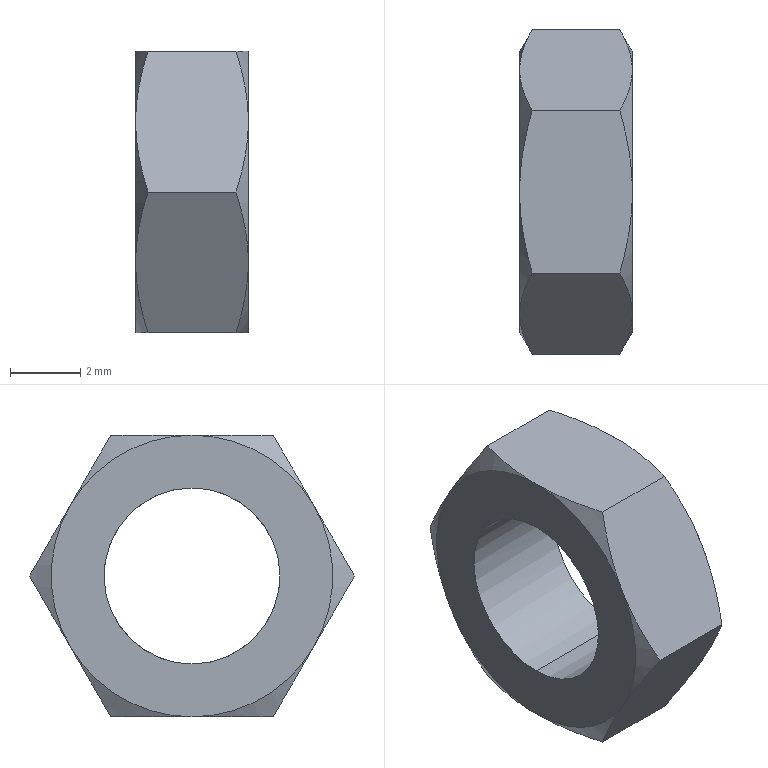Component | SolidWorks | USTH5-15-1_2-1 | 1 solid | 22 faces | box 3.2 x 9.24 x 8 mm | volume 113 mm3 | cone 12 | plane 8 | cylinder 2 | commonest cylinder face diameters 5 x2
STEP:
#1=COLOUR_RGB('',0.7922,0.8196,0.9333);
#2=FILL_AREA_STYLE_COLOUR('',#1);
#3=FILL_AREA_STYLE('',(#2));
#4=SURFACE_STYLE_FILL_AREA(#3);
#5=SURFACE_SIDE_STYLE('',(#4));
#6=SURFACE_STYLE_USAGE(.BOTH.,#5);
#7=PRESENTATION_STYLE_ASSIGNMENT((#6));
#8=CARTESIAN_POINT('',(19.157,0.9252,2.854));
#9=VERTEX_POINT('',#8);
#10=CARTESIAN_POINT('',(19.157,0.9252,3.051));
#11=VERTEX_POINT('',#10);
#12=CARTESIAN_POINT('',(19.157,0.9252,2.953));
#13=DIRECTION('',(-1.,0.,0.));
#14=DIRECTION('',(0.,0.,1.));
#15=AXIS2_PLACEMENT_3D('',#12,#13,#14);
#16=CIRCLE('',#15,0.09843);
#17=EDGE_CURVE('',#9,#11,#16,.T.);
#18=ORIENTED_EDGE('',*,*,#17,.F.);
#19=CARTESIAN_POINT('',(19.031,0.9252,2.854));
#20=VERTEX_POINT('',#19);
#21=CARTESIAN_POINT('',(19.157,0.9252,2.854));
#22=DIRECTION('',(-1.,0.,0.));
#23=VECTOR('',#22,39.37);
#24=LINE('',#21,#23);
#25=EDGE_CURVE('',#9,#20,#24,.T.);
#26=ORIENTED_EDGE('',*,*,#25,.T.);
#27=CARTESIAN_POINT('',(19.031,0.9252,3.051));
#28=VERTEX_POINT('',#27);
#29=CARTESIAN_POINT('',(19.031,0.9252,2.854));
#30=CARTESIAN_POINT('',(19.031,0.9123,2.854));
#31=CARTESIAN_POINT('',(19.031,0.8994,2.857));
#32=CARTESIAN_POINT('',(19.031,0.8756,2.867));
#33=CARTESIAN_POINT('',(19.031,0.8647,2.874));
#34=CARTESIAN_POINT('',(19.031,0.8465,2.892));
#35=CARTESIAN_POINT('',(19.031,0.8392,2.903));
#36=CARTESIAN_POINT('',(19.031,0.8293,2.927));
#37=CARTESIAN_POINT('',(19.031,0.8268,2.94));
#38=CARTESIAN_POINT('',(19.031,0.8268,2.966));
#39=CARTESIAN_POINT('',(19.031,0.8293,2.979));
#40=CARTESIAN_POINT('',(19.031,0.8392,3.002));
#41=CARTESIAN_POINT('',(19.031,0.8465,3.013));
#42=CARTESIAN_POINT('',(19.031,0.8647,3.031));
#43=CARTESIAN_POINT('',(19.031,0.8756,3.039));
#44=CARTESIAN_POINT('',(19.031,0.8994,3.049));
#45=CARTESIAN_POINT('',(19.031,0.9123,3.051));
#46=CARTESIAN_POINT('',(19.031,0.9252,3.051));
#47=B_SPLINE_CURVE_WITH_KNOTS('',3,(#29,#30,#31,#32,#33,#34,#35,#36,#37,#38,#39,#40,#41,#42,#43,#44,#45,#46),.UNSPECIFIED.,.F.,.F.,(4,2,2,2,2,2,2,2,4),(0.5,0.5625,0.625,0.6875,0.75,0.8125,0.875,0.9375,1.),.UNSPECIFIED.);
#48=EDGE_CURVE('',#20,#28,#47,.T.);
#49=ORIENTED_EDGE('',*,*,#48,.T.);
#50=CARTESIAN_POINT('',(19.157,0.9252,3.051));
#51=DIRECTION('',(-1.,0.,0.));
#52=VECTOR('',#51,39.37);
#53=LINE('',#50,#52);
#54=EDGE_CURVE('',#11,#28,#53,.T.);
#55=ORIENTED_EDGE('',*,*,#54,.F.);
#56=EDGE_LOOP('',(#18,#26,#49,#55));
#57=FACE_OUTER_BOUND('',#56,.T.);
#58=CARTESIAN_POINT('',(19.157,0.9252,2.953));
#59=DIRECTION('',(-1.,0.,0.));
#60=DIRECTION('',(0.,0.,1.));
#61=AXIS2_PLACEMENT_3D('',#58,#59,#60);
#62=CYLINDRICAL_SURFACE('',#61,0.09843);
#63=ADVANCED_FACE('',(#57),#62,.F.);
#64=CARTESIAN_POINT('',(19.157,1.062,3.031));
#65=VERTEX_POINT('',#64);
#66=CARTESIAN_POINT('',(19.157,0.9252,3.11));
#67=VERTEX_POINT('',#66);
#68=CARTESIAN_POINT('',(19.157,0.9252,2.953));
#69=DIRECTION('',(1.,0.,0.));
#70=DIRECTION('',(0.,0.,1.));
#71=AXIS2_PLACEMENT_3D('',#68,#69,#70);
#72=CIRCLE('',#71,0.1575);
#73=EDGE_CURVE('',#65,#67,#72,.T.);
#74=ORIENTED_EDGE('',*,*,#73,.T.);
#75=CARTESIAN_POINT('',(19.157,0.7888,3.031));
#76=VERTEX_POINT('',#75);
#77=CARTESIAN_POINT('',(19.157,0.9252,2.953));
#78=DIRECTION('',(1.,0.,0.));
#79=DIRECTION('',(0.,0.,1.));
#80=AXIS2_PLACEMENT_3D('',#77,#78,#79);
#81=CIRCLE('',#80,0.1575);
#82=EDGE_CURVE('',#67,#76,#81,.T.);
#83=ORIENTED_EDGE('',*,*,#82,.T.);
#84=CARTESIAN_POINT('',(19.157,0.7888,2.874));
#85=VERTEX_POINT('',#84);
#86=CARTESIAN_POINT('',(19.157,0.9252,2.953));
#87=DIRECTION('',(1.,0.,0.));
#88=DIRECTION('',(0.,0.,1.));
#89=AXIS2_PLACEMENT_3D('',#86,#87,#88);
#90=CIRCLE('',#89,0.1575);
#91=EDGE_CURVE('',#76,#85,#90,.T.);
#92=ORIENTED_EDGE('',*,*,#91,.T.);
#93=CARTESIAN_POINT('',(19.157,0.9252,2.795));
#94=VERTEX_POINT('',#93);
#95=CARTESIAN_POINT('',(19.157,0.9252,2.953));
#96=DIRECTION('',(1.,0.,0.));
#97=DIRECTION('',(0.,0.,1.));
#98=AXIS2_PLACEMENT_3D('',#95,#96,#97);
#99=CIRCLE('',#98,0.1575);
#100=EDGE_CURVE('',#85,#94,#99,.T.);
#101=ORIENTED_EDGE('',*,*,#100,.T.);
#102=CARTESIAN_POINT('',(19.157,1.062,2.874));
#103=VERTEX_POINT('',#102);
#104=CARTESIAN_POINT('',(19.157,0.9252,2.953));
#105=DIRECTION('',(1.,0.,0.));
#106=DIRECTION('',(0.,-0.,1.));
#107=AXIS2_PLACEMENT_3D('',#104,#105,#106);
#108=CIRCLE('',#107,0.1575);
#109=EDGE_CURVE('',#94,#103,#108,.T.);
#110=ORIENTED_EDGE('',*,*,#109,.T.);
#111=CARTESIAN_POINT('',(19.157,0.9252,2.953));
#112=DIRECTION('',(1.,0.,0.));
#113=DIRECTION('',(0.,0.,1.));
#114=AXIS2_PLACEMENT_3D('',#111,#112,#113);
#115=CIRCLE('',#114,0.1575);
#116=EDGE_CURVE('',#103,#65,#115,.T.);
#117=ORIENTED_EDGE('',*,*,#116,.T.);
#118=EDGE_LOOP('',(#74,#83,#92,#101,#110,#117));
#119=FACE_OUTER_BOUND('',#118,.T.);
#120=CARTESIAN_POINT('',(19.157,0.9252,2.953));
#121=DIRECTION('',(-1.,0.,0.));
#122=DIRECTION('',(0.,0.,1.));
#123=AXIS2_PLACEMENT_3D('',#120,#121,#122);
#124=CIRCLE('',#123,0.09843);
#125=EDGE_CURVE('',#11,#9,#124,.T.);
#126=ORIENTED_EDGE('',*,*,#125,.T.);
#127=ORIENTED_EDGE('',*,*,#17,.T.);
#128=EDGE_LOOP('',(#126,#127));
#129=FACE_BOUND('',#128,.T.);
#130=CARTESIAN_POINT('',(19.157,0.8465,2.953));
#131=DIRECTION('',(1.,0.,0.));
#132=DIRECTION('',(0.,0.,-1.));
#133=AXIS2_PLACEMENT_3D('',#130,#131,#132);
#134=PLANE('',#133);
#135=ADVANCED_FACE('',(#119,#129),#134,.T.);
#136=CARTESIAN_POINT('',(19.143,0.8343,3.11));
#137=VERTEX_POINT('',#136);
#138=CARTESIAN_POINT('',(19.143,0.8343,3.11));
#139=CARTESIAN_POINT('',(19.151,0.8194,3.085));
#140=CARTESIAN_POINT('',(19.157,0.8043,3.058));
#141=CARTESIAN_POINT('',(19.157,0.7888,3.031));
#142=B_SPLINE_CURVE_WITH_KNOTS('',3,(#138,#139,#140,#141),.UNSPECIFIED.,.F.,.F.,(4,4),(0.,0.002337),.UNSPECIFIED.);
#143=EDGE_CURVE('',#137,#76,#142,.T.);
#144=ORIENTED_EDGE('',*,*,#143,.T.);
#145=ORIENTED_EDGE('',*,*,#82,.F.);
#146=CARTESIAN_POINT('',(19.157,0.9252,3.11));
#147=CARTESIAN_POINT('',(19.157,0.8942,3.11));
#148=CARTESIAN_POINT('',(19.151,0.864,3.11));
#149=CARTESIAN_POINT('',(19.143,0.8343,3.11));
#150=B_SPLINE_CURVE_WITH_KNOTS('',3,(#146,#147,#148,#149),.UNSPECIFIED.,.F.,.F.,(4,4),(0.,0.002337),.UNSPECIFIED.);
#151=EDGE_CURVE('',#67,#137,#150,.T.);
#152=ORIENTED_EDGE('',*,*,#151,.T.);
#153=EDGE_LOOP('',(#144,#145,#152));
#154=FACE_OUTER_BOUND('',#153,.T.);
#155=CARTESIAN_POINT('',(19.143,0.9252,2.953));
#156=DIRECTION('',(-1.,0.,0.));
#157=DIRECTION('',(0.,0.,1.));
#158=AXIS2_PLACEMENT_3D('',#155,#156,#157);
#159=CONICAL_SURFACE('',#158,0.182,1.047);
#160=ADVANCED_FACE('',(#154),#159,.T.);
#161=CARTESIAN_POINT('',(19.143,1.016,3.11));
#162=VERTEX_POINT('',#161);
#163=CARTESIAN_POINT('',(19.143,1.016,3.11));
#164=CARTESIAN_POINT('',(19.151,0.9864,3.11));
#165=CARTESIAN_POINT('',(19.157,0.9562,3.11));
#166=CARTESIAN_POINT('',(19.157,0.9252,3.11));
#167=B_SPLINE_CURVE_WITH_KNOTS('',3,(#163,#164,#165,#166),.UNSPECIFIED.,.F.,.F.,(4,4),(0.,0.002337),.UNSPECIFIED.);
#168=EDGE_CURVE('',#162,#67,#167,.T.);
#169=ORIENTED_EDGE('',*,*,#168,.T.);
#170=ORIENTED_EDGE('',*,*,#73,.F.);
#171=CARTESIAN_POINT('',(19.157,1.062,3.031));
#172=CARTESIAN_POINT('',(19.157,1.046,3.058));
#173=CARTESIAN_POINT('',(19.151,1.031,3.085));
#174=CARTESIAN_POINT('',(19.143,1.016,3.11));
#175=B_SPLINE_CURVE_WITH_KNOTS('',3,(#171,#172,#173,#174),.UNSPECIFIED.,.F.,.F.,(4,4),(0.,0.002337),.UNSPECIFIED.);
#176=EDGE_CURVE('',#65,#162,#175,.T.);
#177=ORIENTED_EDGE('',*,*,#176,.T.);
#178=EDGE_LOOP('',(#169,#170,#177));
#179=FACE_OUTER_BOUND('',#178,.T.);
#180=CARTESIAN_POINT('',(19.143,0.9252,2.953));
#181=DIRECTION('',(-1.,0.,0.));
#182=DIRECTION('',(0.,0.,1.));
#183=AXIS2_PLACEMENT_3D('',#180,#181,#182);
#184=CONICAL_SURFACE('',#183,0.182,1.047);
#185=ADVANCED_FACE('',(#179),#184,.T.);
#186=CARTESIAN_POINT('',(19.143,1.107,2.953));
#187=VERTEX_POINT('',#186);
#188=CARTESIAN_POINT('',(19.143,1.107,2.953));
#189=CARTESIAN_POINT('',(19.151,1.092,2.978));
#190=CARTESIAN_POINT('',(19.157,1.077,3.005));
#191=CARTESIAN_POINT('',(19.157,1.062,3.031));
#192=B_SPLINE_CURVE_WITH_KNOTS('',3,(#188,#189,#190,#191),.UNSPECIFIED.,.F.,.F.,(4,4),(0.,0.002337),.UNSPECIFIED.);
#193=EDGE_CURVE('',#187,#65,#192,.T.);
#194=ORIENTED_EDGE('',*,*,#193,.T.);
#195=ORIENTED_EDGE('',*,*,#116,.F.);
#196=CARTESIAN_POINT('',(19.157,1.062,2.874));
#197=CARTESIAN_POINT('',(19.157,1.077,2.901));
#198=CARTESIAN_POINT('',(19.151,1.092,2.927));
#199=CARTESIAN_POINT('',(19.143,1.107,2.953));
#200=B_SPLINE_CURVE_WITH_KNOTS('',3,(#196,#197,#198,#199),.UNSPECIFIED.,.F.,.F.,(4,4),(0.,0.002337),.UNSPECIFIED.);
#201=EDGE_CURVE('',#103,#187,#200,.T.);
#202=ORIENTED_EDGE('',*,*,#201,.T.);
#203=EDGE_LOOP('',(#194,#195,#202));
#204=FACE_OUTER_BOUND('',#203,.T.);
#205=CARTESIAN_POINT('',(19.143,0.9252,2.953));
#206=DIRECTION('',(-1.,0.,0.));
#207=DIRECTION('',(0.,0.,1.));
#208=AXIS2_PLACEMENT_3D('',#205,#206,#207);
#209=CONICAL_SURFACE('',#208,0.182,1.047);
#210=ADVANCED_FACE('',(#204),#209,.T.);
#211=ORIENTED_EDGE('',*,*,#109,.F.);
#212=CARTESIAN_POINT('',(19.143,1.016,2.795));
#213=VERTEX_POINT('',#212);
#214=CARTESIAN_POINT('',(19.157,0.9252,2.795));
#215=CARTESIAN_POINT('',(19.157,0.9562,2.795));
#216=CARTESIAN_POINT('',(19.151,0.9864,2.795));
#217=CARTESIAN_POINT('',(19.143,1.016,2.795));
#218=B_SPLINE_CURVE_WITH_KNOTS('',3,(#214,#215,#216,#217),.UNSPECIFIED.,.F.,.F.,(4,4),(0.,0.002337),.UNSPECIFIED.);
#219=EDGE_CURVE('',#94,#213,#218,.T.);
#220=ORIENTED_EDGE('',*,*,#219,.T.);
#221=CARTESIAN_POINT('',(19.143,1.016,2.795));
#222=CARTESIAN_POINT('',(19.151,1.031,2.821));
#223=CARTESIAN_POINT('',(19.157,1.046,2.847));
#224=CARTESIAN_POINT('',(19.157,1.062,2.874));
#225=B_SPLINE_CURVE_WITH_KNOTS('',3,(#221,#222,#223,#224),.UNSPECIFIED.,.F.,.F.,(4,4),(0.,0.002337),.UNSPECIFIED.);
#226=EDGE_CURVE('',#213,#103,#225,.T.);
#227=ORIENTED_EDGE('',*,*,#226,.T.);
#228=EDGE_LOOP('',(#211,#220,#227));
#229=FACE_OUTER_BOUND('',#228,.T.);
#230=CARTESIAN_POINT('',(19.143,0.9252,2.953));
#231=DIRECTION('',(-1.,0.,0.));
#232=DIRECTION('',(0.,0.,1.));
#233=AXIS2_PLACEMENT_3D('',#230,#231,#232);
#234=CONICAL_SURFACE('',#233,0.182,1.047);
#235=ADVANCED_FACE('',(#229),#234,.T.);
#236=ORIENTED_EDGE('',*,*,#100,.F.);
#237=CARTESIAN_POINT('',(19.143,0.8343,2.795));
#238=VERTEX_POINT('',#237);
#239=CARTESIAN_POINT('',(19.157,0.7888,2.874));
#240=CARTESIAN_POINT('',(19.157,0.8043,2.847));
#241=CARTESIAN_POINT('',(19.151,0.8194,2.821));
#242=CARTESIAN_POINT('',(19.143,0.8343,2.795));
#243=B_SPLINE_CURVE_WITH_KNOTS('',3,(#239,#240,#241,#242),.UNSPECIFIED.,.F.,.F.,(4,4),(0.,0.002337),.UNSPECIFIED.);
#244=EDGE_CURVE('',#85,#238,#243,.T.);
#245=ORIENTED_EDGE('',*,*,#244,.T.);
#246=CARTESIAN_POINT('',(19.143,0.8343,2.795));
#247=CARTESIAN_POINT('',(19.151,0.864,2.795));
#248=CARTESIAN_POINT('',(19.157,0.8942,2.795));
#249=CARTESIAN_POINT('',(19.157,0.9252,2.795));
#250=B_SPLINE_CURVE_WITH_KNOTS('',3,(#246,#247,#248,#249),.UNSPECIFIED.,.F.,.F.,(4,4),(0.,0.002337),.UNSPECIFIED.);
#251=EDGE_CURVE('',#238,#94,#250,.T.);
#252=ORIENTED_EDGE('',*,*,#251,.T.);
#253=EDGE_LOOP('',(#236,#245,#252));
#254=FACE_OUTER_BOUND('',#253,.T.);
#255=CARTESIAN_POINT('',(19.143,0.9252,2.953));
#256=DIRECTION('',(-1.,0.,0.));
#257=DIRECTION('',(0.,0.,1.));
#258=AXIS2_PLACEMENT_3D('',#255,#256,#257);
#259=CONICAL_SURFACE('',#258,0.182,1.047);
#260=ADVANCED_FACE('',(#254),#259,.T.);
#261=CARTESIAN_POINT('',(19.143,0.7434,2.953));
#262=VERTEX_POINT('',#261);
#263=CARTESIAN_POINT('',(19.143,0.7434,2.953));
#264=CARTESIAN_POINT('',(19.151,0.7582,2.927));
#265=CARTESIAN_POINT('',(19.157,0.7733,2.901));
#266=CARTESIAN_POINT('',(19.157,0.7888,2.874));
#267=B_SPLINE_CURVE_WITH_KNOTS('',3,(#263,#264,#265,#266),.UNSPECIFIED.,.F.,.F.,(4,4),(0.,0.002337),.UNSPECIFIED.);
#268=EDGE_CURVE('',#262,#85,#267,.T.);
#269=ORIENTED_EDGE('',*,*,#268,.T.);
#270=ORIENTED_EDGE('',*,*,#91,.F.);
#271=CARTESIAN_POINT('',(19.157,0.7888,3.031));
#272=CARTESIAN_POINT('',(19.157,0.7733,3.005));
#273=CARTESIAN_POINT('',(19.151,0.7582,2.978));
#274=CARTESIAN_POINT('',(19.143,0.7434,2.953));
#275=B_SPLINE_CURVE_WITH_KNOTS('',3,(#271,#272,#273,#274),.UNSPECIFIED.,.F.,.F.,(4,4),(0.,0.002337),.UNSPECIFIED.);
#276=EDGE_CURVE('',#76,#262,#275,.T.);
#277=ORIENTED_EDGE('',*,*,#276,.T.);
#278=EDGE_LOOP('',(#269,#270,#277));
#279=FACE_OUTER_BOUND('',#278,.T.);
#280=CARTESIAN_POINT('',(19.143,0.9252,2.953));
#281=DIRECTION('',(-1.,0.,0.));
#282=DIRECTION('',(0.,0.,1.));
#283=AXIS2_PLACEMENT_3D('',#280,#281,#282);
#284=CONICAL_SURFACE('',#283,0.182,1.047);
#285=ADVANCED_FACE('',(#279),#284,.T.);
#286=CARTESIAN_POINT('',(19.045,0.8343,3.11));
#287=VERTEX_POINT('',#286);
#288=CARTESIAN_POINT('',(18.968,0.8343,3.11));
#289=DIRECTION('',(1.,0.,0.));
#290=VECTOR('',#289,39.37);
#291=LINE('',#288,#290);
#292=EDGE_CURVE('',#287,#137,#291,.T.);
#293=ORIENTED_EDGE('',*,*,#292,.F.);
#294=CARTESIAN_POINT('',(19.031,0.7888,3.031));
#295=VERTEX_POINT('',#294);
#296=CARTESIAN_POINT('',(19.031,0.7888,3.031));
#297=CARTESIAN_POINT('',(19.031,0.8043,3.058));
#298=CARTESIAN_POINT('',(19.036,0.8194,3.085));
#299=CARTESIAN_POINT('',(19.045,0.8343,3.11));
#300=B_SPLINE_CURVE_WITH_KNOTS('',3,(#296,#297,#298,#299),.UNSPECIFIED.,.F.,.F.,(4,4),(0.,0.002337),.UNSPECIFIED.);
#301=EDGE_CURVE('',#295,#287,#300,.T.);
#302=ORIENTED_EDGE('',*,*,#301,.F.);
#303=CARTESIAN_POINT('',(19.045,0.7434,2.953));
#304=VERTEX_POINT('',#303);
#305=CARTESIAN_POINT('',(19.045,0.7434,2.953));
#306=CARTESIAN_POINT('',(19.036,0.7582,2.978));
#307=CARTESIAN_POINT('',(19.031,0.7733,3.005));
#308=CARTESIAN_POINT('',(19.031,0.7888,3.031));
#309=B_SPLINE_CURVE_WITH_KNOTS('',3,(#305,#306,#307,#308),.UNSPECIFIED.,.F.,.F.,(4,4),(0.,0.002337),.UNSPECIFIED.);
#310=EDGE_CURVE('',#304,#295,#309,.T.);
#311=ORIENTED_EDGE('',*,*,#310,.F.);
#312=CARTESIAN_POINT('',(18.968,0.7434,2.953));
#313=DIRECTION('',(-1.,0.,0.));
#314=VECTOR('',#313,39.37);
#315=LINE('',#312,#314);
#316=EDGE_CURVE('',#262,#304,#315,.T.);
#317=ORIENTED_EDGE('',*,*,#316,.F.);
#318=ORIENTED_EDGE('',*,*,#276,.F.);
#319=ORIENTED_EDGE('',*,*,#143,.F.);
#320=EDGE_LOOP('',(#293,#302,#311,#317,#318,#319));
#321=FACE_OUTER_BOUND('',#320,.T.);
#322=CARTESIAN_POINT('',(18.968,0.8343,3.11));
#323=DIRECTION('',(0.,0.866,-0.5));
#324=DIRECTION('',(0.,0.5,0.866));
#325=AXIS2_PLACEMENT_3D('',#322,#323,#324);
#326=PLANE('',#325);
#327=ADVANCED_FACE('',(#321),#326,.F.);
#328=CARTESIAN_POINT('',(19.045,1.016,3.11));
#329=VERTEX_POINT('',#328);
#330=CARTESIAN_POINT('',(18.968,1.016,3.11));
#331=DIRECTION('',(1.,0.,0.));
#332=VECTOR('',#331,39.37);
#333=LINE('',#330,#332);
#334=EDGE_CURVE('',#329,#162,#333,.T.);
#335=ORIENTED_EDGE('',*,*,#334,.F.);
#336=CARTESIAN_POINT('',(19.031,0.9252,3.11));
#337=VERTEX_POINT('',#336);
#338=CARTESIAN_POINT('',(19.031,0.9252,3.11));
#339=CARTESIAN_POINT('',(19.031,0.9562,3.11));
#340=CARTESIAN_POINT('',(19.036,0.9864,3.11));
#341=CARTESIAN_POINT('',(19.045,1.016,3.11));
#342=B_SPLINE_CURVE_WITH_KNOTS('',3,(#338,#339,#340,#341),.UNSPECIFIED.,.F.,.F.,(4,4),(0.,0.002337),.UNSPECIFIED.);
#343=EDGE_CURVE('',#337,#329,#342,.T.);
#344=ORIENTED_EDGE('',*,*,#343,.F.);
#345=CARTESIAN_POINT('',(19.045,0.8343,3.11));
#346=CARTESIAN_POINT('',(19.036,0.864,3.11));
#347=CARTESIAN_POINT('',(19.031,0.8942,3.11));
#348=CARTESIAN_POINT('',(19.031,0.9252,3.11));
#349=B_SPLINE_CURVE_WITH_KNOTS('',3,(#345,#346,#347,#348),.UNSPECIFIED.,.F.,.F.,(4,4),(0.,0.002337),.UNSPECIFIED.);
#350=EDGE_CURVE('',#287,#337,#349,.T.);
#351=ORIENTED_EDGE('',*,*,#350,.F.);
#352=ORIENTED_EDGE('',*,*,#292,.T.);
#353=ORIENTED_EDGE('',*,*,#151,.F.);
#354=ORIENTED_EDGE('',*,*,#168,.F.);
#355=EDGE_LOOP('',(#335,#344,#351,#352,#353,#354));
#356=FACE_OUTER_BOUND('',#355,.T.);
#357=CARTESIAN_POINT('',(18.968,1.016,3.11));
#358=DIRECTION('',(0.,0.,-1.));
#359=DIRECTION('',(-1.,0.,0.));
#360=AXIS2_PLACEMENT_3D('',#357,#358,#359);
#361=PLANE('',#360);
#362=ADVANCED_FACE('',(#356),#361,.F.);
#363=CARTESIAN_POINT('',(19.045,1.107,2.953));
#364=VERTEX_POINT('',#363);
#365=CARTESIAN_POINT('',(18.968,1.107,2.953));
#366=DIRECTION('',(1.,0.,0.));
#367=VECTOR('',#366,39.37);
#368=LINE('',#365,#367);
#369=EDGE_CURVE('',#364,#187,#368,.T.);
#370=ORIENTED_EDGE('',*,*,#369,.F.);
#371=CARTESIAN_POINT('',(19.031,1.062,3.031));
#372=VERTEX_POINT('',#371);
#373=CARTESIAN_POINT('',(19.031,1.062,3.031));
#374=CARTESIAN_POINT('',(19.031,1.077,3.005));
#375=CARTESIAN_POINT('',(19.036,1.092,2.978));
#376=CARTESIAN_POINT('',(19.045,1.107,2.953));
#377=B_SPLINE_CURVE_WITH_KNOTS('',3,(#373,#374,#375,#376),.UNSPECIFIED.,.F.,.F.,(4,4),(0.,0.002337),.UNSPECIFIED.);
#378=EDGE_CURVE('',#372,#364,#377,.T.);
#379=ORIENTED_EDGE('',*,*,#378,.F.);
#380=CARTESIAN_POINT('',(19.045,1.016,3.11));
#381=CARTESIAN_POINT('',(19.036,1.031,3.085));
#382=CARTESIAN_POINT('',(19.031,1.046,3.058));
#383=CARTESIAN_POINT('',(19.031,1.062,3.031));
#384=B_SPLINE_CURVE_WITH_KNOTS('',3,(#380,#381,#382,#383),.UNSPECIFIED.,.F.,.F.,(4,4),(0.,0.002337),.UNSPECIFIED.);
#385=EDGE_CURVE('',#329,#372,#384,.T.);
#386=ORIENTED_EDGE('',*,*,#385,.F.);
#387=ORIENTED_EDGE('',*,*,#334,.T.);
#388=ORIENTED_EDGE('',*,*,#176,.F.);
#389=ORIENTED_EDGE('',*,*,#193,.F.);
#390=EDGE_LOOP('',(#370,#379,#386,#387,#388,#389));
#391=FACE_OUTER_BOUND('',#390,.T.);
#392=CARTESIAN_POINT('',(18.968,1.107,2.953));
#393=DIRECTION('',(0.,-0.866,-0.5));
#394=DIRECTION('',(0.,0.5,-0.866));
#395=AXIS2_PLACEMENT_3D('',#392,#393,#394);
#396=PLANE('',#395);
#397=ADVANCED_FACE('',(#391),#396,.F.);
#398=ORIENTED_EDGE('',*,*,#226,.F.);
#399=CARTESIAN_POINT('',(19.045,1.016,2.795));
#400=VERTEX_POINT('',#399);
#401=CARTESIAN_POINT('',(18.968,1.016,2.795));
#402=DIRECTION('',(1.,0.,0.));
#403=VECTOR('',#402,39.37);
#404=LINE('',#401,#403);
#405=EDGE_CURVE('',#400,#213,#404,.T.);
#406=ORIENTED_EDGE('',*,*,#405,.F.);
#407=CARTESIAN_POINT('',(19.031,1.062,2.874));
#408=VERTEX_POINT('',#407);
#409=CARTESIAN_POINT('',(19.031,1.062,2.874));
#410=CARTESIAN_POINT('',(19.031,1.046,2.847));
#411=CARTESIAN_POINT('',(19.036,1.031,2.821));
#412=CARTESIAN_POINT('',(19.045,1.016,2.795));
#413=B_SPLINE_CURVE_WITH_KNOTS('',3,(#409,#410,#411,#412),.UNSPECIFIED.,.F.,.F.,(4,4),(0.,0.002337),.UNSPECIFIED.);
#414=EDGE_CURVE('',#408,#400,#413,.T.);
#415=ORIENTED_EDGE('',*,*,#414,.F.);
#416=CARTESIAN_POINT('',(19.045,1.107,2.953));
#417=CARTESIAN_POINT('',(19.036,1.092,2.927));
#418=CARTESIAN_POINT('',(19.031,1.077,2.901));
#419=CARTESIAN_POINT('',(19.031,1.062,2.874));
#420=B_SPLINE_CURVE_WITH_KNOTS('',3,(#416,#417,#418,#419),.UNSPECIFIED.,.F.,.F.,(4,4),(0.,0.002337),.UNSPECIFIED.);
#421=EDGE_CURVE('',#364,#408,#420,.T.);
#422=ORIENTED_EDGE('',*,*,#421,.F.);
#423=ORIENTED_EDGE('',*,*,#369,.T.);
#424=ORIENTED_EDGE('',*,*,#201,.F.);
#425=EDGE_LOOP('',(#398,#406,#415,#422,#423,#424));
#426=FACE_OUTER_BOUND('',#425,.T.);
#427=CARTESIAN_POINT('',(18.968,1.016,2.795));
#428=DIRECTION('',(0.,-0.866,0.5));
#429=DIRECTION('',(0.,-0.5,-0.866));
#430=AXIS2_PLACEMENT_3D('',#427,#428,#429);
#431=PLANE('',#430);
#432=ADVANCED_FACE('',(#426),#431,.F.);
#433=ORIENTED_EDGE('',*,*,#251,.F.);
#434=CARTESIAN_POINT('',(19.045,0.8343,2.795));
#435=VERTEX_POINT('',#434);
#436=CARTESIAN_POINT('',(18.968,0.8343,2.795));
#437=DIRECTION('',(1.,0.,0.));
#438=VECTOR('',#437,39.37);
#439=LINE('',#436,#438);
#440=EDGE_CURVE('',#435,#238,#439,.T.);
#441=ORIENTED_EDGE('',*,*,#440,.F.);
#442=CARTESIAN_POINT('',(19.031,0.9252,2.795));
#443=VERTEX_POINT('',#442);
#444=CARTESIAN_POINT('',(19.031,0.9252,2.795));
#445=CARTESIAN_POINT('',(19.031,0.8942,2.795));
#446=CARTESIAN_POINT('',(19.036,0.864,2.795));
#447=CARTESIAN_POINT('',(19.045,0.8343,2.795));
#448=B_SPLINE_CURVE_WITH_KNOTS('',3,(#444,#445,#446,#447),.UNSPECIFIED.,.F.,.F.,(4,4),(0.,0.002337),.UNSPECIFIED.);
#449=EDGE_CURVE('',#443,#435,#448,.T.);
#450=ORIENTED_EDGE('',*,*,#449,.F.);
#451=CARTESIAN_POINT('',(19.045,1.016,2.795));
#452=CARTESIAN_POINT('',(19.036,0.9864,2.795));
#453=CARTESIAN_POINT('',(19.031,0.9562,2.795));
#454=CARTESIAN_POINT('',(19.031,0.9252,2.795));
#455=B_SPLINE_CURVE_WITH_KNOTS('',3,(#451,#452,#453,#454),.UNSPECIFIED.,.F.,.F.,(4,4),(0.,0.002337),.UNSPECIFIED.);
#456=EDGE_CURVE('',#400,#443,#455,.T.);
#457=ORIENTED_EDGE('',*,*,#456,.F.);
#458=ORIENTED_EDGE('',*,*,#405,.T.);
#459=ORIENTED_EDGE('',*,*,#219,.F.);
#460=EDGE_LOOP('',(#433,#441,#450,#457,#458,#459));
#461=FACE_OUTER_BOUND('',#460,.T.);
#462=CARTESIAN_POINT('',(18.968,0.8343,2.795));
#463=DIRECTION('',(0.,0.,1.));
#464=DIRECTION('',(1.,0.,0.));
#465=AXIS2_PLACEMENT_3D('',#462,#463,#464);
#466=PLANE('',#465);
#467=ADVANCED_FACE('',(#461),#466,.F.);
#468=ORIENTED_EDGE('',*,*,#268,.F.);
#469=ORIENTED_EDGE('',*,*,#316,.T.);
#470=CARTESIAN_POINT('',(19.031,0.7888,2.874));
#471=VERTEX_POINT('',#470);
#472=CARTESIAN_POINT('',(19.031,0.7888,2.874));
#473=CARTESIAN_POINT('',(19.031,0.7733,2.901));
#474=CARTESIAN_POINT('',(19.036,0.7582,2.927));
#475=CARTESIAN_POINT('',(19.045,0.7434,2.953));
#476=B_SPLINE_CURVE_WITH_KNOTS('',3,(#472,#473,#474,#475),.UNSPECIFIED.,.F.,.F.,(4,4),(0.,0.002337),.UNSPECIFIED.);
#477=EDGE_CURVE('',#471,#304,#476,.T.);
#478=ORIENTED_EDGE('',*,*,#477,.F.);
#479=CARTESIAN_POINT('',(19.045,0.8343,2.795));
#480=CARTESIAN_POINT('',(19.036,0.8194,2.821));
#481=CARTESIAN_POINT('',(19.031,0.8043,2.847));
#482=CARTESIAN_POINT('',(19.031,0.7888,2.874));
#483=B_SPLINE_CURVE_WITH_KNOTS('',3,(#479,#480,#481,#482),.UNSPECIFIED.,.F.,.F.,(4,4),(0.,0.002337),.UNSPECIFIED.);
#484=EDGE_CURVE('',#435,#471,#483,.T.);
#485=ORIENTED_EDGE('',*,*,#484,.F.);
#486=ORIENTED_EDGE('',*,*,#440,.T.);
#487=ORIENTED_EDGE('',*,*,#244,.F.);
#488=EDGE_LOOP('',(#468,#469,#478,#485,#486,#487));
#489=FACE_OUTER_BOUND('',#488,.T.);
#490=CARTESIAN_POINT('',(18.968,0.7434,2.953));
#491=DIRECTION('',(0.,0.866,0.5));
#492=DIRECTION('',(0.,-0.5,0.866));
#493=AXIS2_PLACEMENT_3D('',#490,#491,#492);
#494=PLANE('',#493);
#495=ADVANCED_FACE('',(#489),#494,.F.);
#496=ORIENTED_EDGE('',*,*,#350,.T.);
#497=CARTESIAN_POINT('',(19.031,0.9252,2.953));
#498=DIRECTION('',(1.,0.,0.));
#499=DIRECTION('',(0.,0.,-1.));
#500=AXIS2_PLACEMENT_3D('',#497,#498,#499);
#501=CIRCLE('',#500,0.1575);
#502=EDGE_CURVE('',#337,#295,#501,.T.);
#503=ORIENTED_EDGE('',*,*,#502,.T.);
#504=ORIENTED_EDGE('',*,*,#301,.T.);
#505=EDGE_LOOP('',(#496,#503,#504));
#506=FACE_OUTER_BOUND('',#505,.T.);
#507=CARTESIAN_POINT('',(19.045,0.9252,2.953));
#508=DIRECTION('',(1.,0.,0.));
#509=DIRECTION('',(0.,0.,-1.));
#510=AXIS2_PLACEMENT_3D('',#507,#508,#509);
#511=CONICAL_SURFACE('',#510,0.182,1.047);
#512=ADVANCED_FACE('',(#506),#511,.T.);
#513=ORIENTED_EDGE('',*,*,#310,.T.);
#514=CARTESIAN_POINT('',(19.031,0.9252,2.953));
#515=DIRECTION('',(1.,0.,0.));
#516=DIRECTION('',(0.,0.,-1.));
#517=AXIS2_PLACEMENT_3D('',#514,#515,#516);
#518=CIRCLE('',#517,0.1575);
#519=EDGE_CURVE('',#295,#471,#518,.T.);
#520=ORIENTED_EDGE('',*,*,#519,.T.);
#521=ORIENTED_EDGE('',*,*,#477,.T.);
#522=EDGE_LOOP('',(#513,#520,#521));
#523=FACE_OUTER_BOUND('',#522,.T.);
#524=CARTESIAN_POINT('',(19.045,0.9252,2.953));
#525=DIRECTION('',(1.,0.,0.));
#526=DIRECTION('',(0.,0.,-1.));
#527=AXIS2_PLACEMENT_3D('',#524,#525,#526);
#528=CONICAL_SURFACE('',#527,0.182,1.047);
#529=ADVANCED_FACE('',(#523),#528,.T.);
#530=CARTESIAN_POINT('',(19.031,0.9252,2.953));
#531=DIRECTION('',(1.,0.,0.));
#532=DIRECTION('',(0.,0.,-1.));
#533=AXIS2_PLACEMENT_3D('',#530,#531,#532);
#534=CIRCLE('',#533,0.1575);
#535=EDGE_CURVE('',#372,#337,#534,.T.);
#536=ORIENTED_EDGE('',*,*,#535,.T.);
#537=ORIENTED_EDGE('',*,*,#343,.T.);
#538=ORIENTED_EDGE('',*,*,#385,.T.);
#539=EDGE_LOOP('',(#536,#537,#538));
#540=FACE_OUTER_BOUND('',#539,.T.);
#541=CARTESIAN_POINT('',(19.045,0.9252,2.953));
#542=DIRECTION('',(1.,0.,0.));
#543=DIRECTION('',(0.,0.,-1.));
#544=AXIS2_PLACEMENT_3D('',#541,#542,#543);
#545=CONICAL_SURFACE('',#544,0.182,1.047);
#546=ADVANCED_FACE('',(#540),#545,.T.);
#547=CARTESIAN_POINT('',(19.031,0.9252,2.953));
#548=DIRECTION('',(1.,0.,0.));
#549=DIRECTION('',(0.,0.,-1.));
#550=AXIS2_PLACEMENT_3D('',#547,#548,#549);
#551=CIRCLE('',#550,0.1575);
#552=EDGE_CURVE('',#408,#372,#551,.T.);
#553=ORIENTED_EDGE('',*,*,#552,.T.);
#554=ORIENTED_EDGE('',*,*,#378,.T.);
#555=ORIENTED_EDGE('',*,*,#421,.T.);
#556=EDGE_LOOP('',(#553,#554,#555));
#557=FACE_OUTER_BOUND('',#556,.T.);
#558=CARTESIAN_POINT('',(19.045,0.9252,2.953));
#559=DIRECTION('',(1.,0.,0.));
#560=DIRECTION('',(0.,0.,-1.));
#561=AXIS2_PLACEMENT_3D('',#558,#559,#560);
#562=CONICAL_SURFACE('',#561,0.182,1.047);
#563=ADVANCED_FACE('',(#557),#562,.T.);
#564=CARTESIAN_POINT('',(19.031,0.9252,2.953));
#565=DIRECTION('',(1.,0.,0.));
#566=DIRECTION('',(0.,0.,-1.));
#567=AXIS2_PLACEMENT_3D('',#564,#565,#566);
#568=CIRCLE('',#567,0.1575);
#569=EDGE_CURVE('',#443,#408,#568,.T.);
#570=ORIENTED_EDGE('',*,*,#569,.T.);
#571=ORIENTED_EDGE('',*,*,#414,.T.);
#572=ORIENTED_EDGE('',*,*,#456,.T.);
#573=EDGE_LOOP('',(#570,#571,#572));
#574=FACE_OUTER_BOUND('',#573,.T.);
#575=CARTESIAN_POINT('',(19.045,0.9252,2.953));
#576=DIRECTION('',(1.,0.,0.));
#577=DIRECTION('',(0.,0.,-1.));
#578=AXIS2_PLACEMENT_3D('',#575,#576,#577);
#579=CONICAL_SURFACE('',#578,0.182,1.047);
#580=ADVANCED_FACE('',(#574),#579,.T.);
#581=ORIENTED_EDGE('',*,*,#484,.T.);
#582=CARTESIAN_POINT('',(19.031,0.9252,2.953));
#583=DIRECTION('',(1.,0.,0.));
#584=DIRECTION('',(0.,0.,-1.));
#585=AXIS2_PLACEMENT_3D('',#582,#583,#584);
#586=CIRCLE('',#585,0.1575);
#587=EDGE_CURVE('',#471,#443,#586,.T.);
#588=ORIENTED_EDGE('',*,*,#587,.T.);
#589=ORIENTED_EDGE('',*,*,#449,.T.);
#590=EDGE_LOOP('',(#581,#588,#589));
#591=FACE_OUTER_BOUND('',#590,.T.);
#592=CARTESIAN_POINT('',(19.045,0.9252,2.953));
#593=DIRECTION('',(1.,0.,0.));
#594=DIRECTION('',(0.,0.,-1.));
#595=AXIS2_PLACEMENT_3D('',#592,#593,#594);
#596=CONICAL_SURFACE('',#595,0.182,1.047);
#597=ADVANCED_FACE('',(#591),#596,.T.);
#598=ORIENTED_EDGE('',*,*,#587,.F.);
#599=ORIENTED_EDGE('',*,*,#519,.F.);
#600=ORIENTED_EDGE('',*,*,#502,.F.);
#601=ORIENTED_EDGE('',*,*,#535,.F.);
#602=ORIENTED_EDGE('',*,*,#552,.F.);
#603=ORIENTED_EDGE('',*,*,#569,.F.);
#604=EDGE_LOOP('',(#598,#599,#600,#601,#602,#603));
#605=FACE_OUTER_BOUND('',#604,.T.);
#606=CARTESIAN_POINT('',(19.031,0.9252,3.051));
#607=CARTESIAN_POINT('',(19.031,0.9381,3.051));
#608=CARTESIAN_POINT('',(19.031,0.951,3.049));
#609=CARTESIAN_POINT('',(19.031,0.9748,3.039));
#610=CARTESIAN_POINT('',(19.031,0.9857,3.031));
#611=CARTESIAN_POINT('',(19.031,1.004,3.013));
#612=CARTESIAN_POINT('',(19.031,1.011,3.002));
#613=CARTESIAN_POINT('',(19.031,1.021,2.979));
#614=CARTESIAN_POINT('',(19.031,1.024,2.966));
#615=CARTESIAN_POINT('',(19.031,1.024,2.94));
#616=CARTESIAN_POINT('',(19.031,1.021,2.927));
#617=CARTESIAN_POINT('',(19.031,1.011,2.903));
#618=CARTESIAN_POINT('',(19.031,1.004,2.892));
#619=CARTESIAN_POINT('',(19.031,0.9857,2.874));
#620=CARTESIAN_POINT('',(19.031,0.9748,2.867));
#621=CARTESIAN_POINT('',(19.031,0.951,2.857));
#622=CARTESIAN_POINT('',(19.031,0.9381,2.854));
#623=CARTESIAN_POINT('',(19.031,0.9252,2.854));
#624=B_SPLINE_CURVE_WITH_KNOTS('',3,(#606,#607,#608,#609,#610,#611,#612,#613,#614,#615,#616,#617,#618,#619,#620,#621,#622,#623),.UNSPECIFIED.,.F.,.F.,(4,2,2,2,2,2,2,2,4),(0.,0.0625,0.125,0.1875,0.25,0.3125,0.375,0.4375,0.5),.UNSPECIFIED.);
#625=EDGE_CURVE('',#28,#20,#624,.T.);
#626=ORIENTED_EDGE('',*,*,#625,.F.);
#627=ORIENTED_EDGE('',*,*,#48,.F.);
#628=EDGE_LOOP('',(#626,#627));
#629=FACE_BOUND('',#628,.T.);
#630=CARTESIAN_POINT('',(19.031,0.8465,2.953));
#631=DIRECTION('',(-1.,0.,0.));
#632=DIRECTION('',(0.,0.,1.));
#633=AXIS2_PLACEMENT_3D('',#630,#631,#632);
#634=PLANE('',#633);
#635=ADVANCED_FACE('',(#605,#629),#634,.T.);
#636=ORIENTED_EDGE('',*,*,#25,.F.);
#637=ORIENTED_EDGE('',*,*,#125,.F.);
#638=ORIENTED_EDGE('',*,*,#54,.T.);
#639=ORIENTED_EDGE('',*,*,#625,.T.);
#640=EDGE_LOOP('',(#636,#637,#638,#639));
#641=FACE_OUTER_BOUND('',#640,.T.);
#642=CARTESIAN_POINT('',(19.157,0.9252,2.953));
#643=DIRECTION('',(-1.,0.,0.));
#644=DIRECTION('',(0.,0.,1.));
#645=AXIS2_PLACEMENT_3D('',#642,#643,#644);
#646=CYLINDRICAL_SURFACE('',#645,0.09843);
#647=ADVANCED_FACE('',(#641),#646,.F.);
#648=CLOSED_SHELL('',(#63,#135,#160,#185,#210,#235,#260,#285,#327,#362,#397,#432,#467,#495,#512,#529,#546,#563,#580,#597,#635,#647));
#649=MANIFOLD_SOLID_BREP('',#648);
#650=STYLED_ITEM('',(#7),#649);
#651=(LENGTH_UNIT()NAMED_UNIT(*)SI_UNIT($,.METRE.));
#652=LENGTH_MEASURE_WITH_UNIT(LENGTH_MEASURE(0.0254),#651);
#653=DIMENSIONAL_EXPONENTS(1.,0.,0.,0.,0.,0.,0.);
#654=(CONVERSION_BASED_UNIT('',#652)LENGTH_UNIT()NAMED_UNIT(#653));
#655=UNCERTAINTY_MEASURE_WITH_UNIT(LENGTH_MEASURE(0.00001),#654,'','');
#656=(NAMED_UNIT(*)PLANE_ANGLE_UNIT()SI_UNIT($,.RADIAN.));
#657=(NAMED_UNIT(*)SI_UNIT($,.STERADIAN.)SOLID_ANGLE_UNIT());
#658=(GEOMETRIC_REPRESENTATION_CONTEXT(3)GLOBAL_UNCERTAINTY_ASSIGNED_CONTEXT((#655))GLOBAL_UNIT_ASSIGNED_CONTEXT((#654,#656,#657))REPRESENTATION_CONTEXT('',''));
#659=MECHANICAL_DESIGN_GEOMETRIC_PRESENTATION_REPRESENTATION('',(#650),#658);
#660=CARTESIAN_POINT('',(0.,0.,0.));
#661=DIRECTION('',(0.,0.,1.));
#662=DIRECTION('',(1.,0.,0.));
#663=AXIS2_PLACEMENT_3D('',#660,#661,#662);
#664=(LENGTH_UNIT()NAMED_UNIT(*)SI_UNIT($,.METRE.));
#665=LENGTH_MEASURE_WITH_UNIT(LENGTH_MEASURE(0.0254),#664);
#666=DIMENSIONAL_EXPONENTS(1.,0.,0.,0.,0.,0.,0.);
#667=(CONVERSION_BASED_UNIT('',#665)LENGTH_UNIT()NAMED_UNIT(#666));
#668=UNCERTAINTY_MEASURE_WITH_UNIT(LENGTH_MEASURE(0.00001),#667,'','');
#669=(NAMED_UNIT(*)PLANE_ANGLE_UNIT()SI_UNIT($,.RADIAN.));
#670=(NAMED_UNIT(*)SI_UNIT($,.STERADIAN.)SOLID_ANGLE_UNIT());
#671=(GEOMETRIC_REPRESENTATION_CONTEXT(3)GLOBAL_UNCERTAINTY_ASSIGNED_CONTEXT((#668))GLOBAL_UNIT_ASSIGNED_CONTEXT((#667,#669,#670))REPRESENTATION_CONTEXT('',''));
#672=ADVANCED_BREP_SHAPE_REPRESENTATION('',(#649,#663),#671);
#673=PRESENTATION_LAYER_ASSIGNMENT('','',(#650));